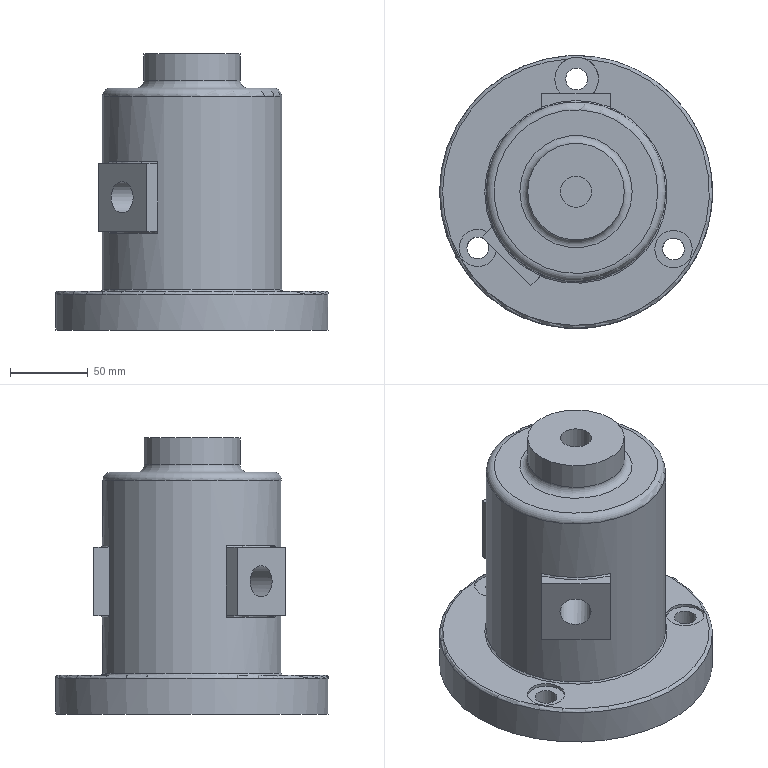Component | NX | VALVE_SEAT | 1 solid | 46 faces | volume 1720636 mm3 | plane 20 | cylinder 15 | torus 8 | cone 3 | commonest cylinder face diameters 20 x3 14 x3 24 x2 175 x1 115 x1 82 x1 62 x1 18 x1